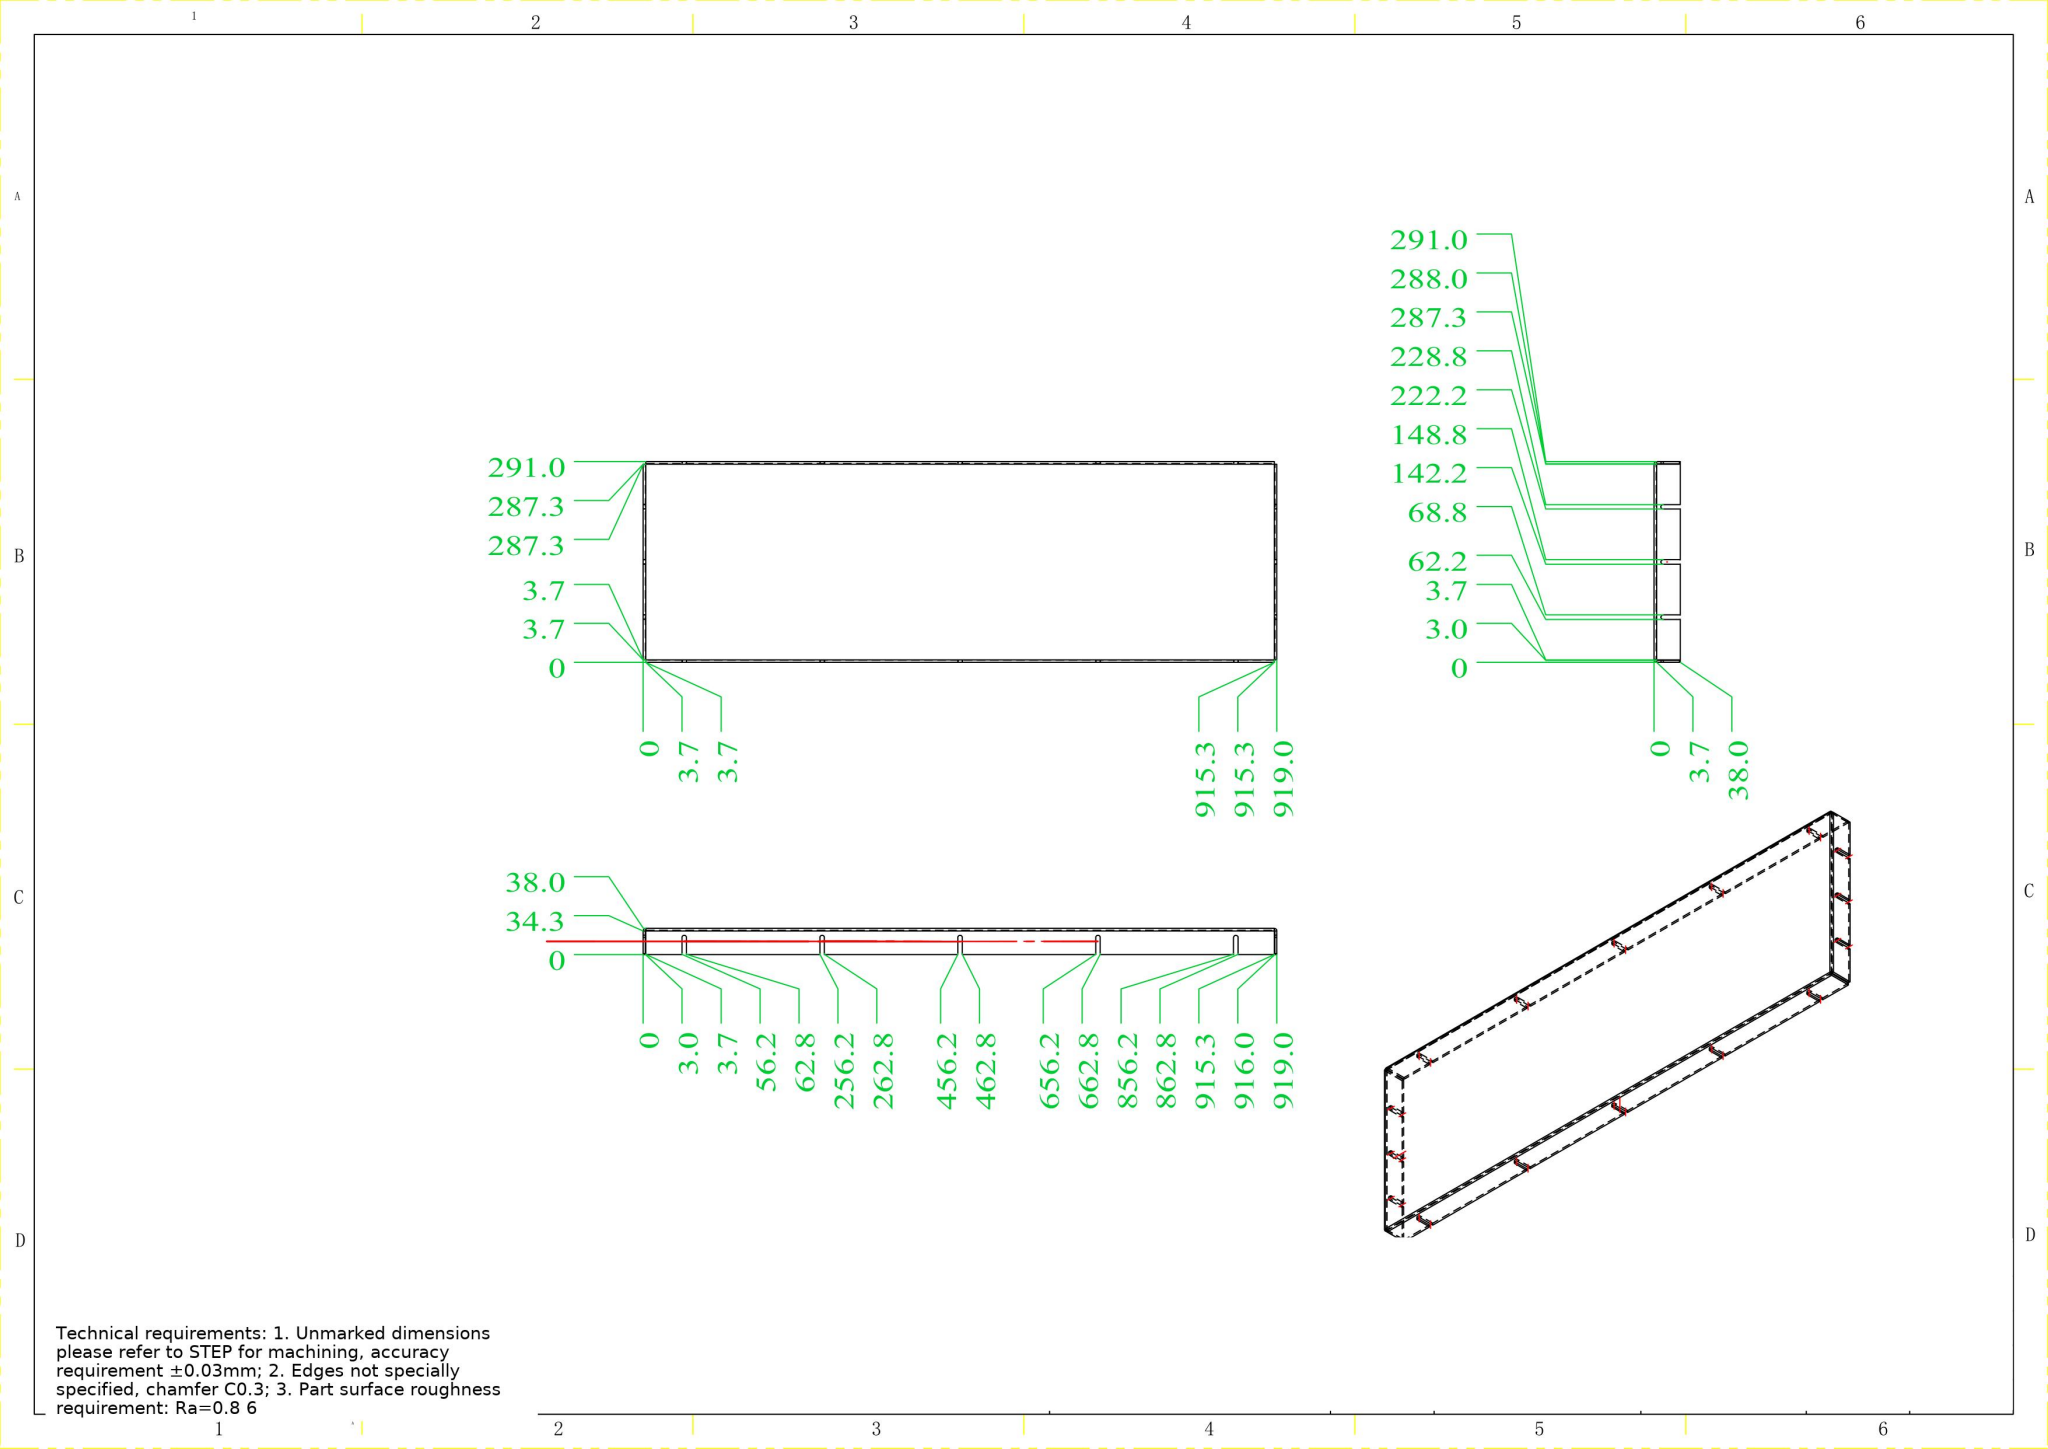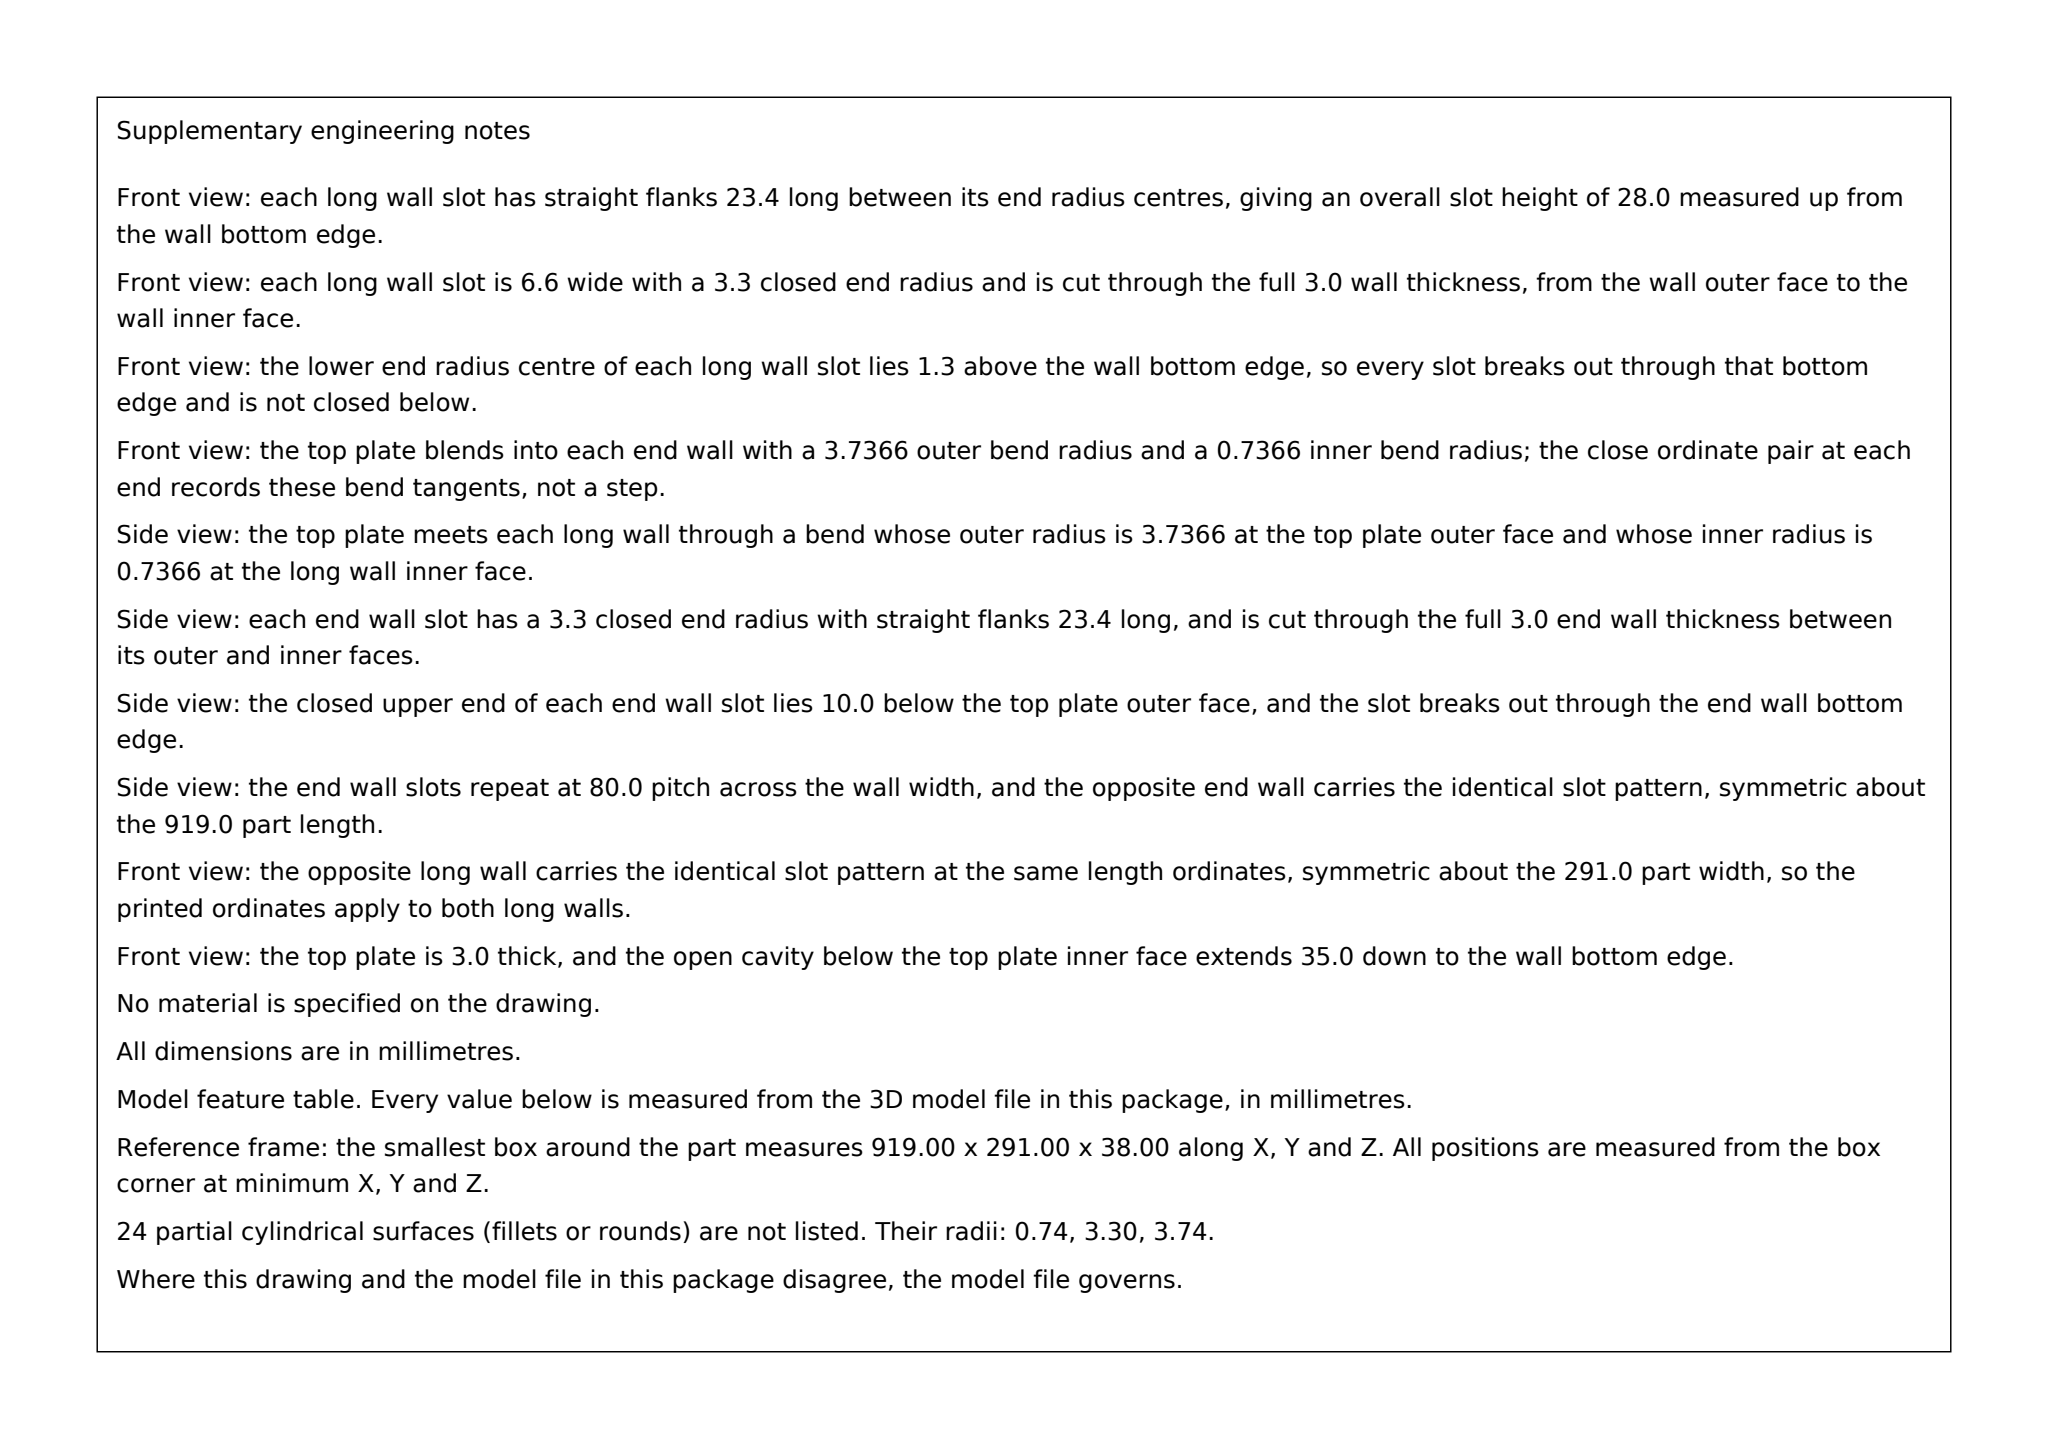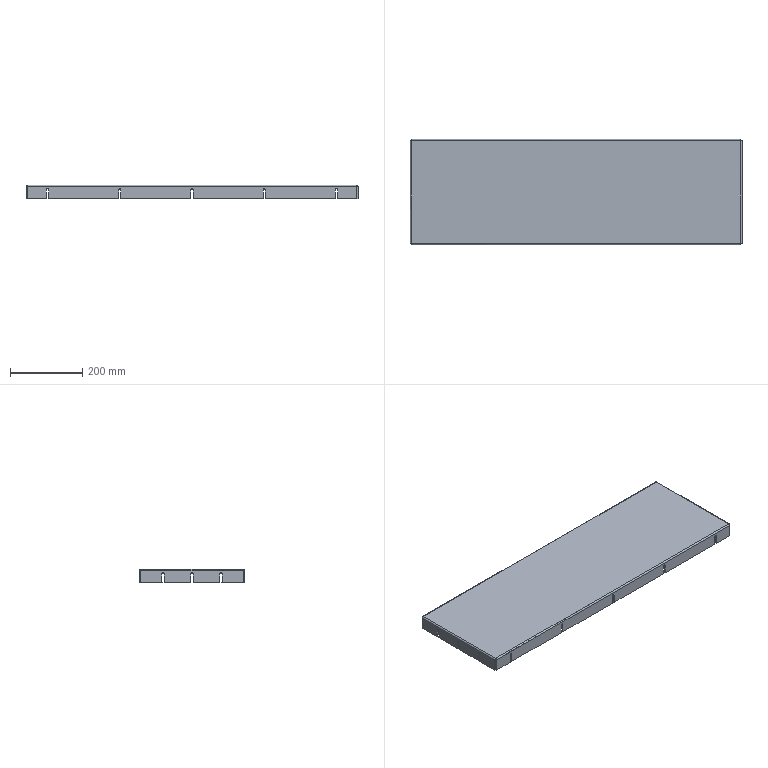Part | SolidWorks | mm | 1 solid | 142 faces | box 919 x 291 x 38 mm | volume 1037588 mm3 | plane 70 | cylinder 64 | spline 8 | commonest cylinder face diameters 6.6 x56 7.473 x4 1.473 x4
Drawing notes:
SLOT 6.6 W: END ARC CTRS Z1.3 & Z24.7, OPEN THRU BTM Z0 | from the solid: 6.6 dia cylinders at z=1.3 and z=24.7, z-plane at 0.0 (20 faces)
ALL 6.6 W SLOTS: R3.3 FULL RAD ENDS, O/A LG 30.0 | from the solid: 6.6 dia end cylinders, ctr spacing 24.7-1.3=23.4 +6.6 = 30.0
CONT GROOVE PROFILE: Ø7.473 W/ Ø1.473 ROOT, CL Z34.26 | from the solid: cylinders dia 7.473 & 1.473, axes at z=34.26, 3.77/287.29/915.29 offsets
GROOVE CL 3.7 FROM EDGE ALL AROUND, LG 911.6 X 283.6 | from the solid: groove axes at x/y 3.77 & 915.29/287.29, lengths 911.59 and 283.59
STEP BELOW 38.0 TOP FACE: 3.0 DP TO Z35.0 FACE | from the solid: z-planes at 38.0 and 35.0; 38.0-35.0=3.0
(1) 3.0 = WALL THK; (2) 28.0 = SLOT TOP END FROM Z0 FACE | from the solid: x-planes 0.03 & 3.03 (3.0 wall); slot top = 24.7+3.3 = 28.0